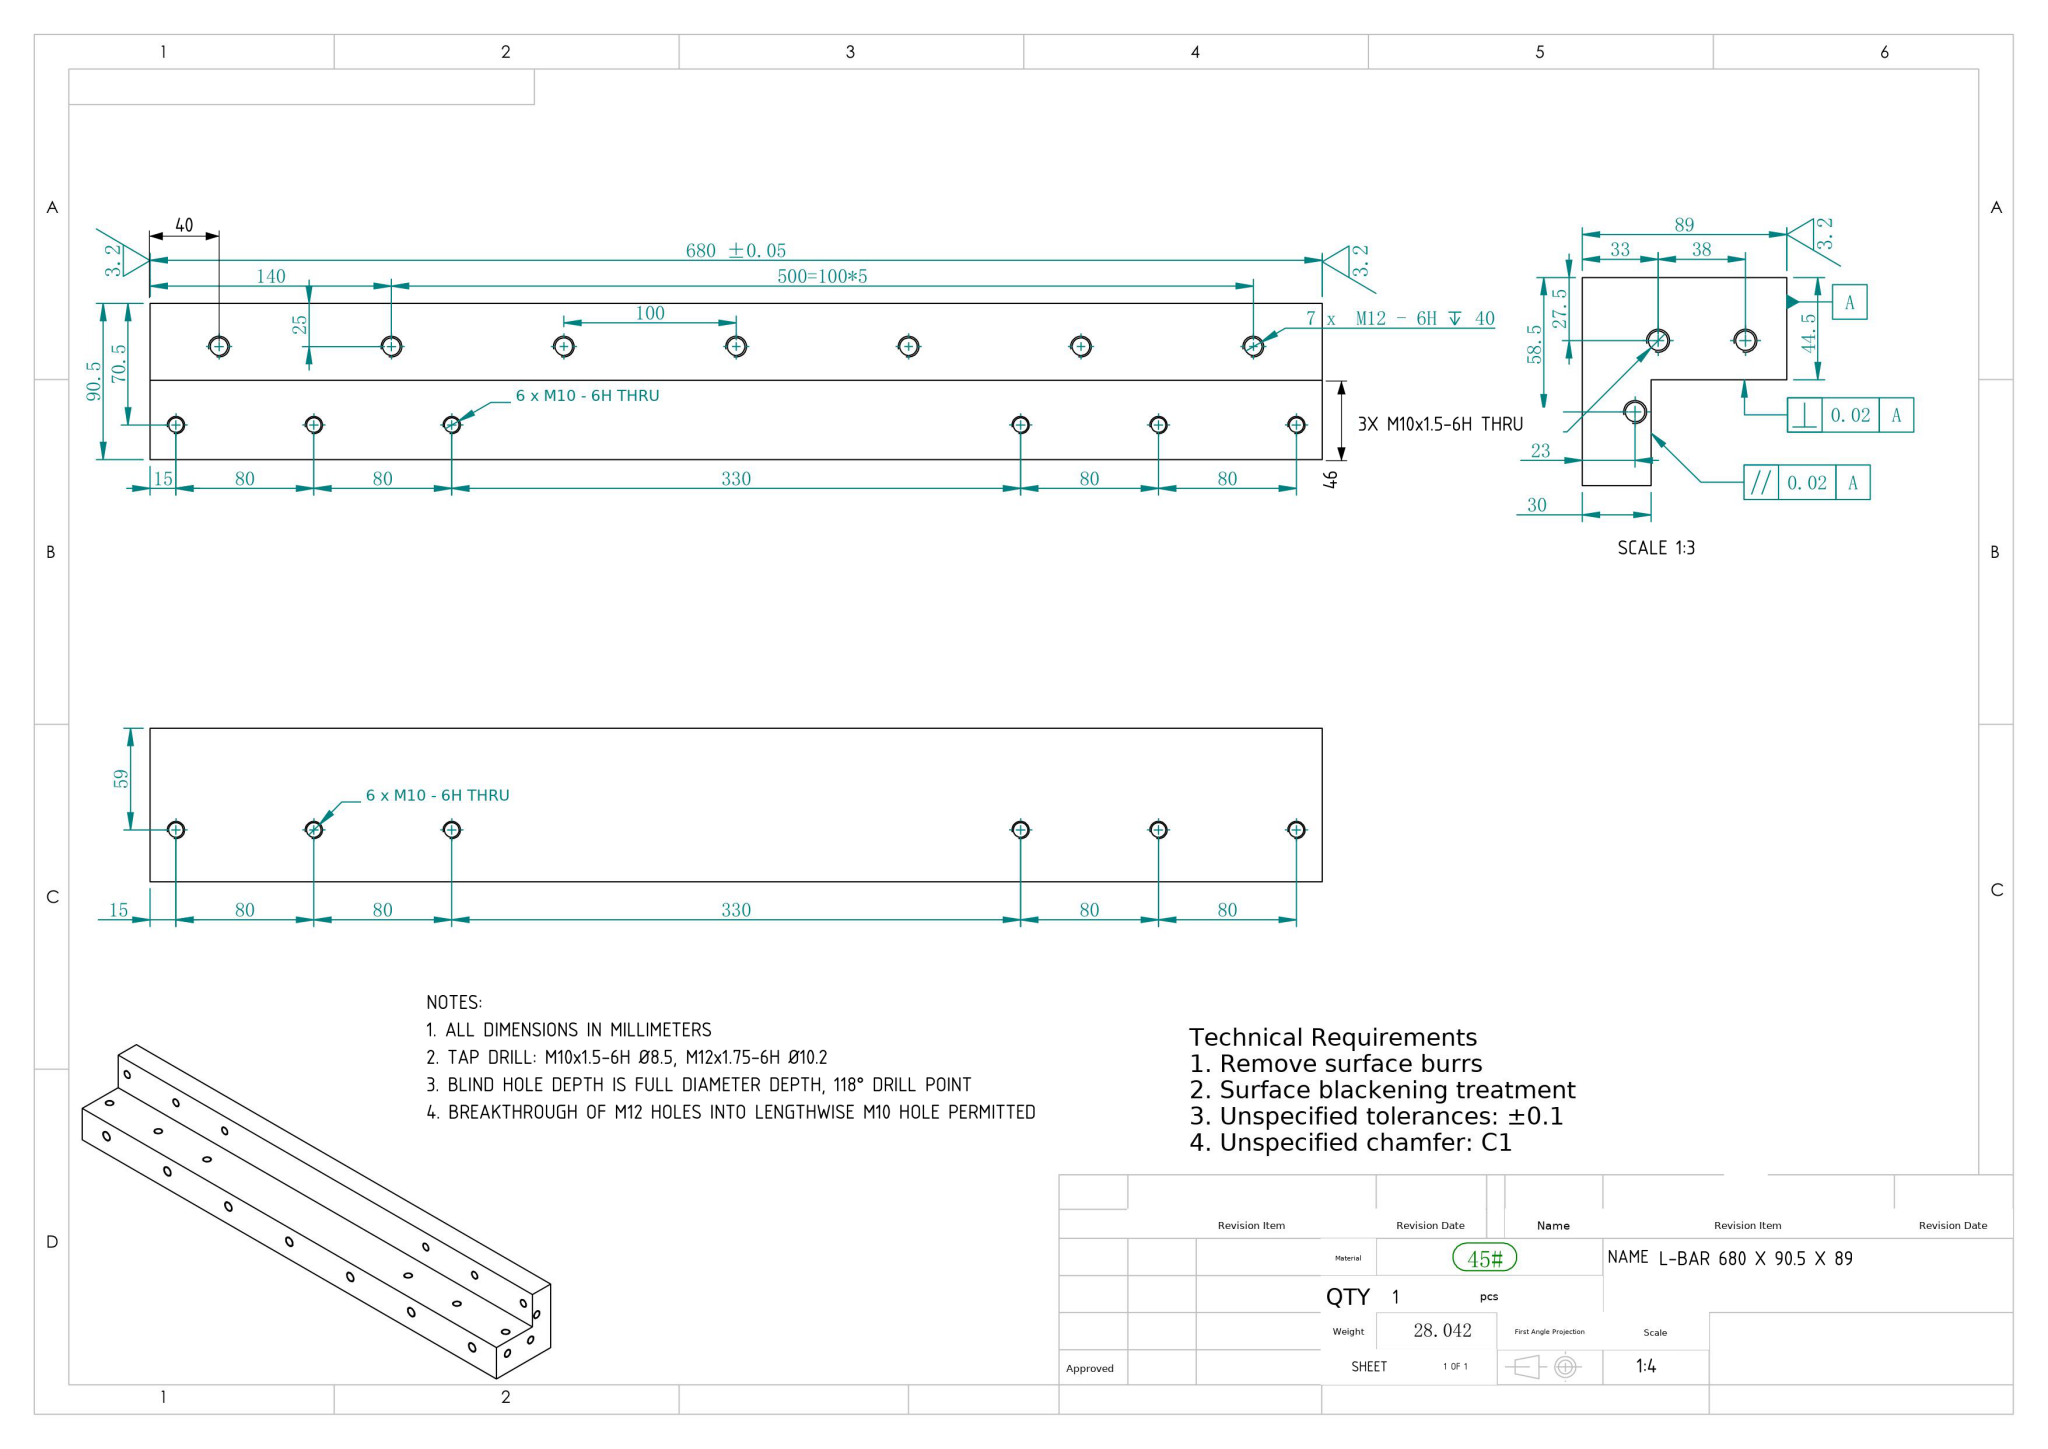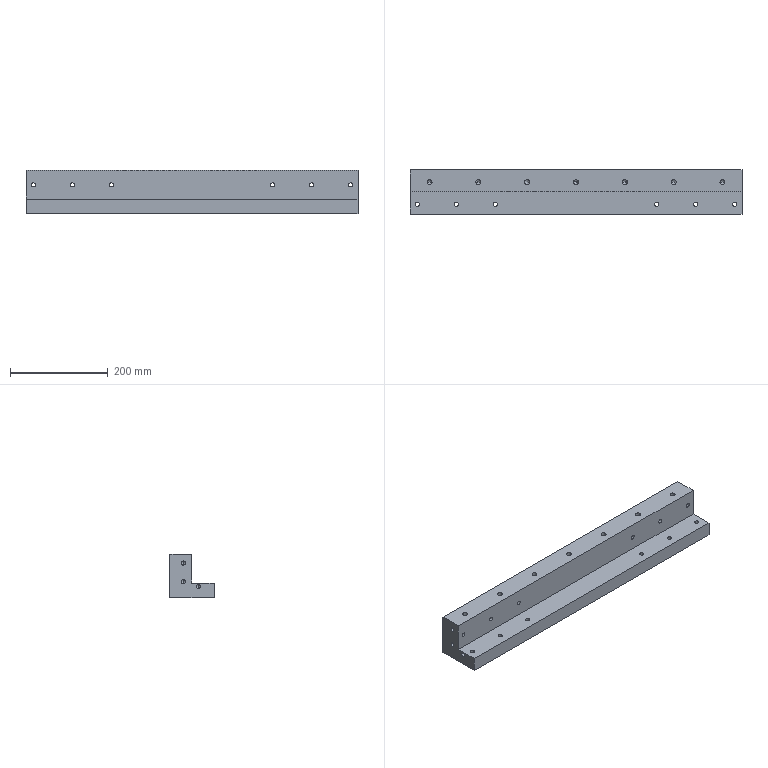Part | NX | mm | 1 solid | 84 faces | box 680 x 90.5 x 89 mm | volume 3572207 mm3 | cylinder 50 | cone 26 | plane 8 | commonest cylinder face diameters 8.5 x36 10.2 x14